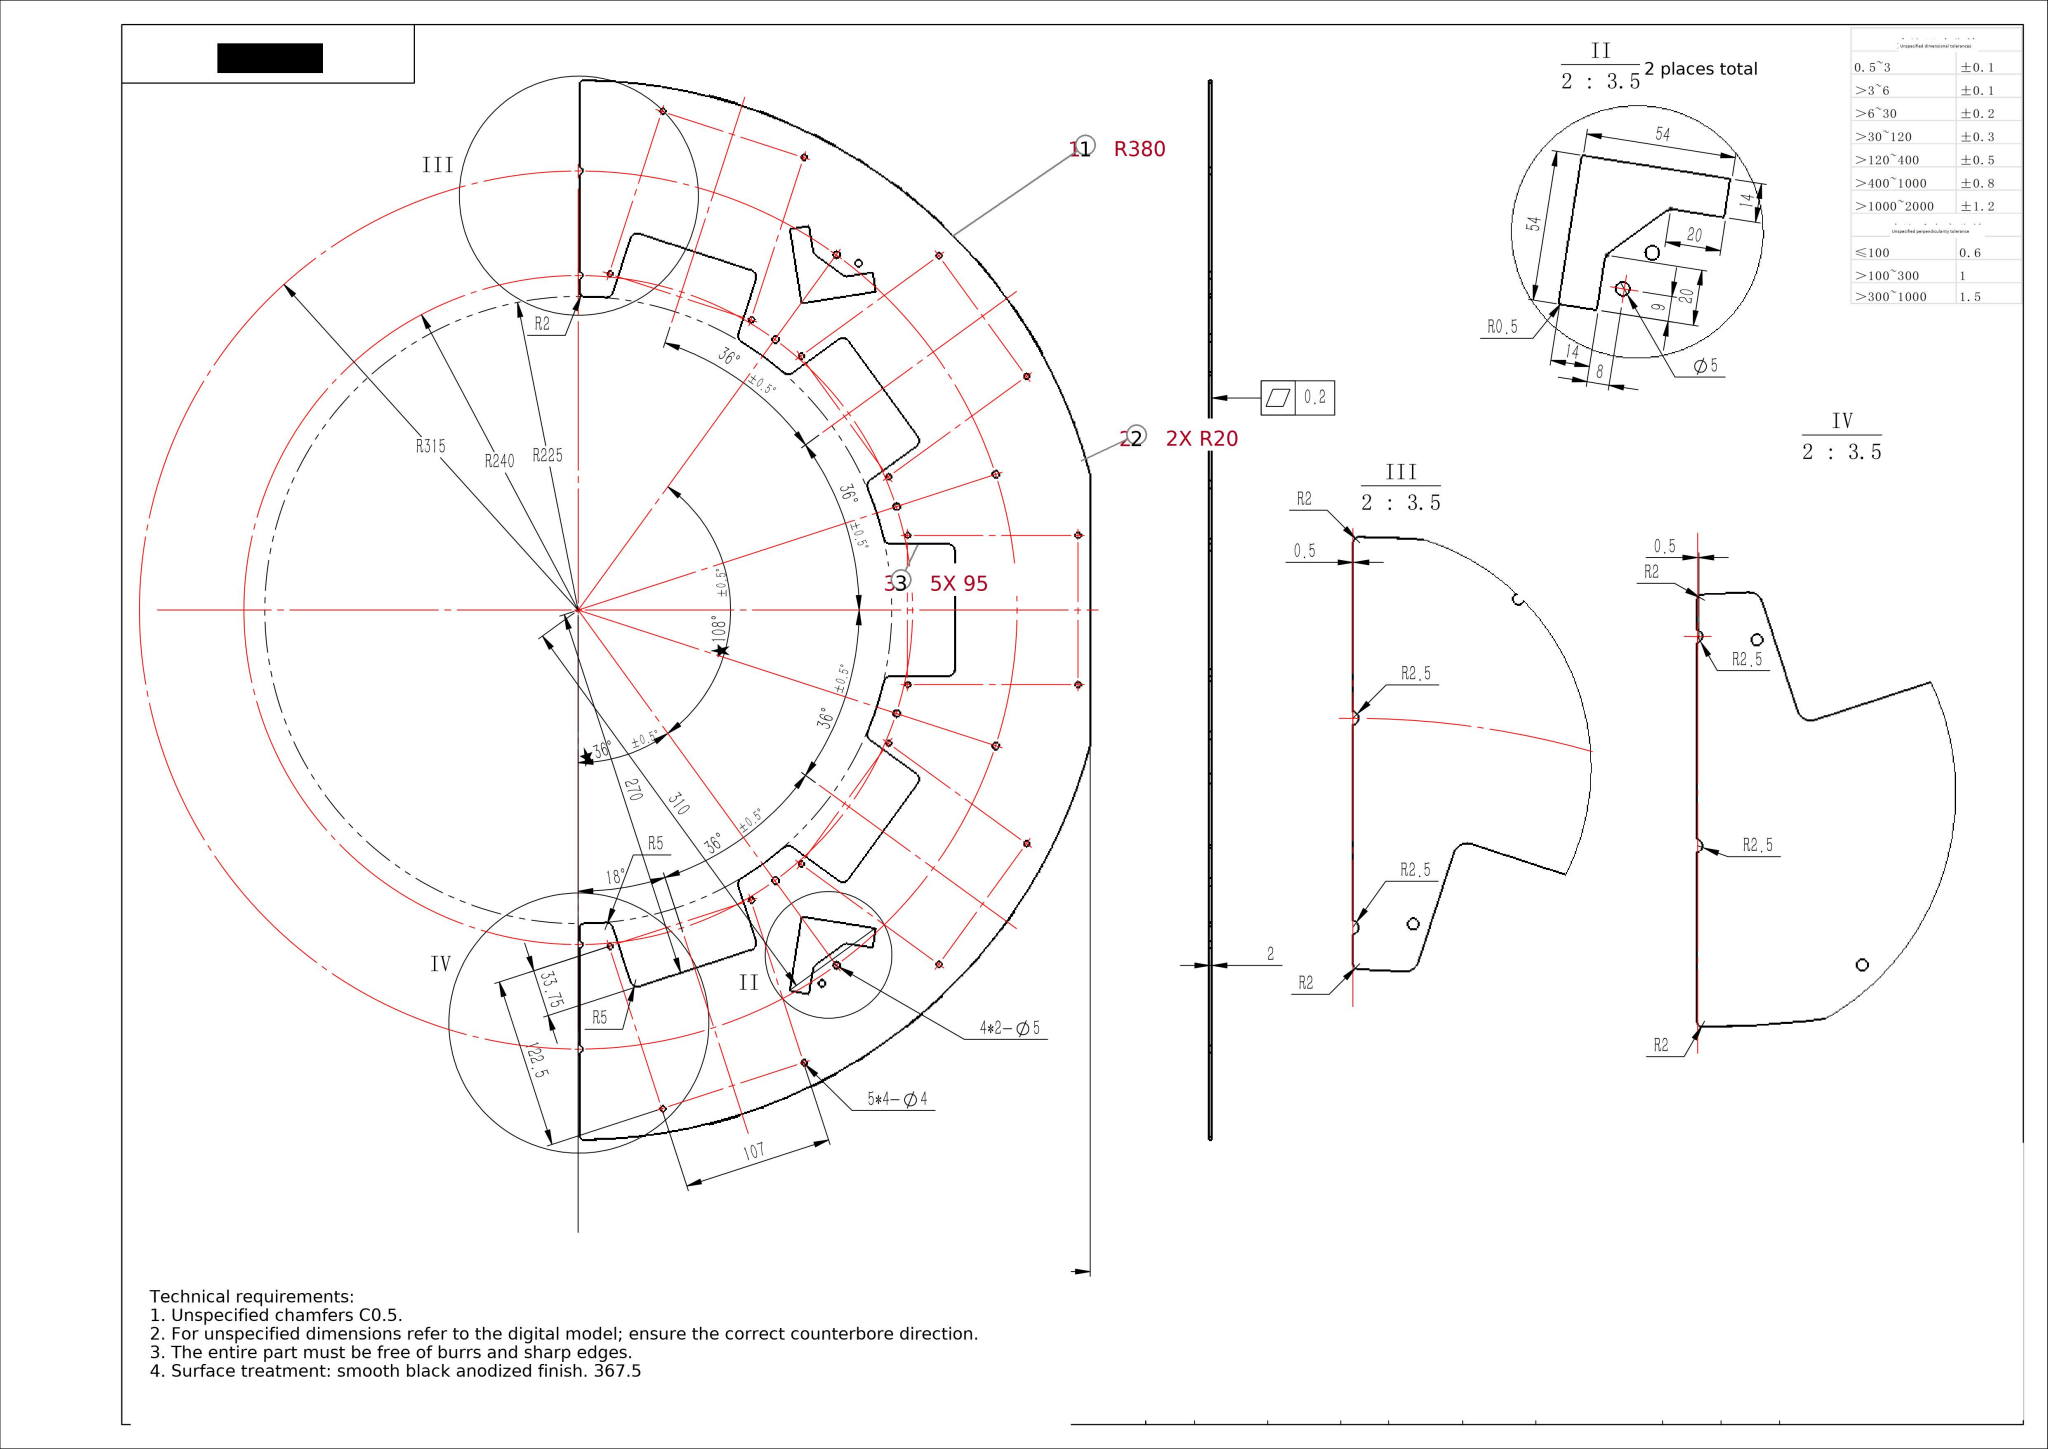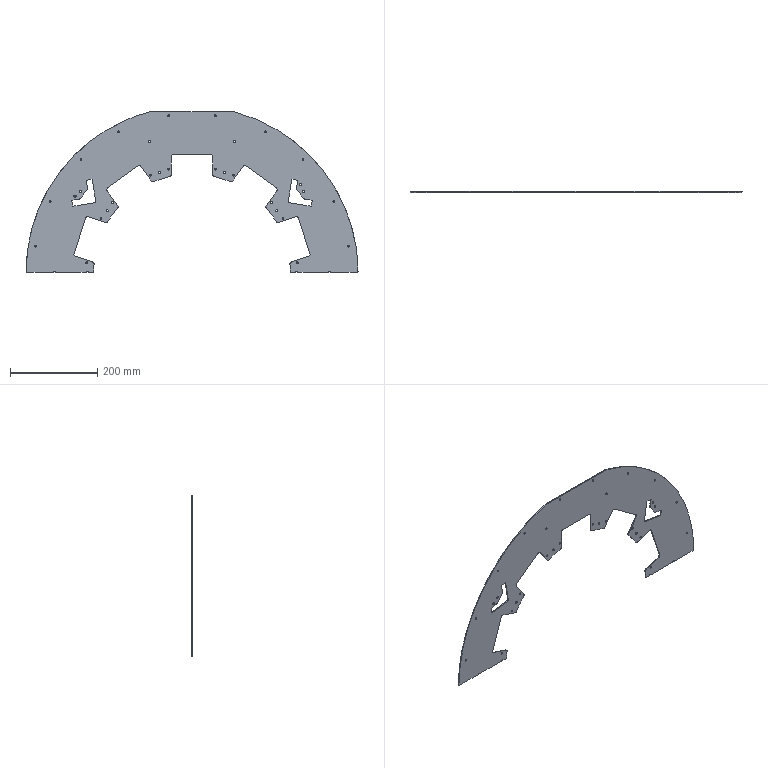Part | SolidWorks | mm | 1 solid | 156 faces | box 759.98 x 2 x 367 mm | volume 239727 mm3 | cylinder 118 | plane 38 | commonest cylinder face diameters 4 x44 5 x28 10 x24 1 x12 450 x6 760 x2 40 x2
build123d program:
from build123d import *

# Parameters (mm, degrees)
BOSS_EXTRUDE1_DEPTH = 2
SKETCH7_W           = 760
SKETCH7_H           = 0.5
CUT_EXTRUDE5_DEPTH  = 538.405
SKETCH8_R           = 2.5
CUT_EXTRUDE6_DEPTH  = 538.405
CUT_EXTRUDE7_DEPTH  = 538.405
SKETCH10_R          = 225
CUT_EXTRUDE8_DEPTH  = 10
CIRPATTERN1_COUNT   = 10
SKETCH11_R          = 2
CUT_EXTRUDE9_DEPTH  = 10
CIRPATTERN2_COUNT   = 10
CIRPATTERN3_COUNT   = 10
FILLET1_R           = 5
FILLET2_R           = 2
SKETCH13_W          = 500
SKETCH13_H          = 25
CUT_EXTRUDE11_DEPTH = 10
FILLET3_R           = 20
CUT_EXTRUDE13_DEPTH = 10
FILLET4_R           = 0.5
FILLET5_R           = 5
SKETCH17_R          = 2.5
CUT_EXTRUDE14_DEPTH = 10
CUT_EXTRUDE15_DEPTH = 10
FILLET6_R           = 5


with BuildPart() as part:
    # Sketch2 → Boss-Extrude1 (new body)
    with BuildSketch(Plane(origin=(0, 0, 0), x_dir=(1, 0, 0), z_dir=(0, 1, 0))):
        with BuildLine():
            Line((-380, 0), (380, 0))
            ThreePointArc((380, 0), (0, -380), (-380, 0))
        make_face()
    extrude(amount=BOSS_EXTRUDE1_DEPTH)

    # Sketch7 → Cut-Extrude5 (cut, through all)
    with BuildSketch(Plane(origin=(0, 2, 0), x_dir=(1, 0, 0), z_dir=(0, 1, 0))):
        with Locations((0, -0.25)):
            Rectangle(SKETCH7_W, SKETCH7_H)
    extrude(amount=-CUT_EXTRUDE5_DEPTH, mode=Mode.SUBTRACT)

    # Sketch8 → Cut-Extrude6 (cut, through all)
    with BuildSketch(Plane(origin=(0, 2, 0), x_dir=(1, 0, 0), z_dir=(0, 1, 0))):
        with Locations((-240, 0)):
            Circle(SKETCH8_R)
        with Locations((-315, 0)):
            Circle(SKETCH8_R)
    cut_extrude6 = extrude(amount=-CUT_EXTRUDE6_DEPTH, mode=Mode.SUBTRACT)

    # Sketch9 → Cut-Extrude7 (cut, through all)
    with BuildSketch(Plane(origin=(0, 2, 0), x_dir=(1, 0, 0), z_dir=(0, 1, 0))):
        Polygon((-271.464, -38.259), (-96.295, 18.656), (-66.939, -71.694), (-242.107, -128.61), align=None)
    cut_extrude7 = extrude(amount=-CUT_EXTRUDE7_DEPTH, mode=Mode.SUBTRACT)

    # Sketch10 → Cut-Extrude8 (cut)
    with BuildSketch(Plane(origin=(0, 2, 0), x_dir=(1, 0, 0), z_dir=(0, 1, 0))):
        Circle(SKETCH10_R)
    extrude(amount=-CUT_EXTRUDE8_DEPTH, mode=Mode.SUBTRACT)

    # CirPattern1: Cut-Extrude7 ×10 about axis
    cirpattern1_axis = Axis((0, 2, 0), (0, -1, 0))
    for i in range(1, CIRPATTERN1_COUNT):
        add(cut_extrude7.rotate(cirpattern1_axis, i * 360 / CIRPATTERN1_COUNT), mode=Mode.SUBTRACT)

    # Sketch11 → Cut-Extrude9 (cut)
    with BuildSketch(Plane(origin=(0, 2, 0), x_dir=(1, 0, 0), z_dir=(0, 1, 0))):
        with Locations(Location((-241.22, -22.124, 0), (0, 0, 270))):
            Circle(SKETCH11_R)
        with Locations(Location((-357.724, -59.978, 0), (0, 0, 270))):
            Circle(SKETCH11_R)
        with Locations(Location((-208.155, -123.887, 0), (0, 0, 270))):
            Circle(SKETCH11_R)
        with Locations(Location((-324.659, -161.741, 0), (0, 0, 270))):
            Circle(SKETCH11_R)
    cut_extrude9 = extrude(amount=-CUT_EXTRUDE9_DEPTH, mode=Mode.SUBTRACT)

    # CirPattern2: Cut-Extrude9 ×10 about axis
    cirpattern2_axis = Axis((0, 2, 0), (0, -1, 0))
    for i in range(1, CIRPATTERN2_COUNT):
        add(cut_extrude9.rotate(cirpattern2_axis, i * 360 / CIRPATTERN2_COUNT), mode=Mode.SUBTRACT)

    # CirPattern3: Cut-Extrude6 ×10 about axis
    cirpattern3_axis = Axis((0, 2, 0), (0, -1, 0))
    for i in range(1, CIRPATTERN3_COUNT):
        add(cut_extrude6.rotate(cirpattern3_axis, i * 360 / CIRPATTERN3_COUNT), mode=Mode.SUBTRACT)

    # Fillet1
    fillet1_edges = [part.edges().sort_by_distance(p)[0] for p in [
        (271.464, 1, 38.259),
        (197.13, 1, 190.515),
        (47.5, 1, 270),
        (-120.274, 1, 246.354),
        (242.107, 1, 128.61),
        (120.274, 1, 246.354),
        (-47.5, 1, 270),
        (-197.13, 1, 190.515),
        (-242.107, 1, 128.61),
        (-271.464, 1, 38.259),
        (-194.487, 1, 113.137),
        (-223.843, 1, 22.787),
        (-90.843, 1, 205.846),
        (-167.699, 1, 150.006),
        (47.5, 1, 219.929),
        (-47.5, 1, 219.929),
        (167.699, 1, 150.006),
        (90.843, 1, 205.846),
        (223.843, 1, 22.787),
        (194.487, 1, 113.137),
    ]]
    fillet(fillet1_edges, radius=FILLET1_R)

    # Fillet2
    fillet2_edges = [part.edges().sort_by_distance(p)[0] for p in [
        (224.999, 1, 0.5),
        (-224.999, 1, 0.5),
        (-380, 1, 0.5),
        (380, 1, 0.5),
    ]]
    fillet(fillet2_edges, radius=FILLET2_R)

    # Sketch13 → Cut-Extrude11 (cut)
    with BuildSketch(Plane(origin=(0, 2, 0), x_dir=(1, 0, 0), z_dir=(0, 1, 0))):
        with Locations((0, -380)):
            Rectangle(SKETCH13_W, SKETCH13_H)
    extrude(amount=-CUT_EXTRUDE11_DEPTH, mode=Mode.SUBTRACT)

    # Fillet3
    fillet3_edges = [part.edges().sort_by_distance(p)[0] for p in [
        (-96.663, 1, 367.5),
        (96.663, 1, 367.5),
    ]]
    fillet(fillet3_edges, radius=FILLET3_R)

    # Sketch16 → Cut-Extrude13 (cut)
    with BuildSketch(Plane(origin=(0, 2, 0), x_dir=(1, 0, 0), z_dir=(0, 1, 0))):
        Polygon((-273.239, -151.322), (-219.904, -159.77), (-228.351, -213.105), (-242.179, -210.915), (-235.922, -171.407), (-275.429, -165.15), align=None)
    cut_extrude13 = extrude(amount=-CUT_EXTRUDE13_DEPTH, mode=Mode.SUBTRACT)

    # Mirror2: Cut-Extrude13 across plane
    add(cut_extrude13.mirror(Plane(origin=(0, 0, 0), x_dir=(0, 0, 1), z_dir=(1, 0, 0))), mode=Mode.SUBTRACT)

    # Fillet4
    fillet4_edges = [part.edges().sort_by_distance(p)[0] for p in [
        (-275.429, 1, 165.15),
        (-273.239, 1, 151.322),
        (-219.904, 1, 159.77),
        (-228.351, 1, 213.105),
        (-242.179, 1, 210.915),
        (273.239, 1, 151.322),
        (275.429, 1, 165.15),
        (242.179, 1, 210.915),
        (228.351, 1, 213.105),
        (219.904, 1, 159.77),
    ]]
    fillet(fillet4_edges, radius=FILLET4_R)

    # Fillet5
    fillet5_edges = [part.edges().sort_by_distance(p)[0] for p in [
        (-235.922, 1, 171.407),
        (235.922, 1, 171.407),
    ]]
    fillet(fillet5_edges, radius=FILLET5_R)

    # Sketch17 → Cut-Extrude14 (cut)
    with BuildSketch(Plane(origin=(0, 2, 0), x_dir=(1, 0, 0), z_dir=(0, 1, 0))):
        with Locations(Location((-267.791, -174.459, 0), (0, 0, 270))):
            Circle(SKETCH17_R)
        with Locations(Location((248.673, -200.774, 0), (0, 0, 270))):
            Circle(SKETCH17_R)
    extrude(amount=-CUT_EXTRUDE14_DEPTH, mode=Mode.SUBTRACT)

    # Sketch18 → Cut-Extrude15 (cut)
    with BuildSketch(Plane(origin=(0, 2, 0), x_dir=(1, 0, 0), z_dir=(0, 1, 0))):
        Polygon((255.675, -168.278), (235.922, -171.407), (239.05, -191.161), align=None)
        Polygon((-255.675, -168.278), (-235.922, -171.407), (-239.05, -191.161), align=None)
    extrude(amount=-CUT_EXTRUDE15_DEPTH, mode=Mode.SUBTRACT)

    # Fillet6
    fillet6_edges = [part.edges().sort_by_distance(p)[0] for p in [
        (255.675, 1, 168.278),
        (239.05, 1, 191.161),
        (-239.05, 1, 191.161),
        (-255.675, 1, 168.278),
    ]]
    fillet(fillet6_edges, radius=FILLET6_R)


solid = part.part